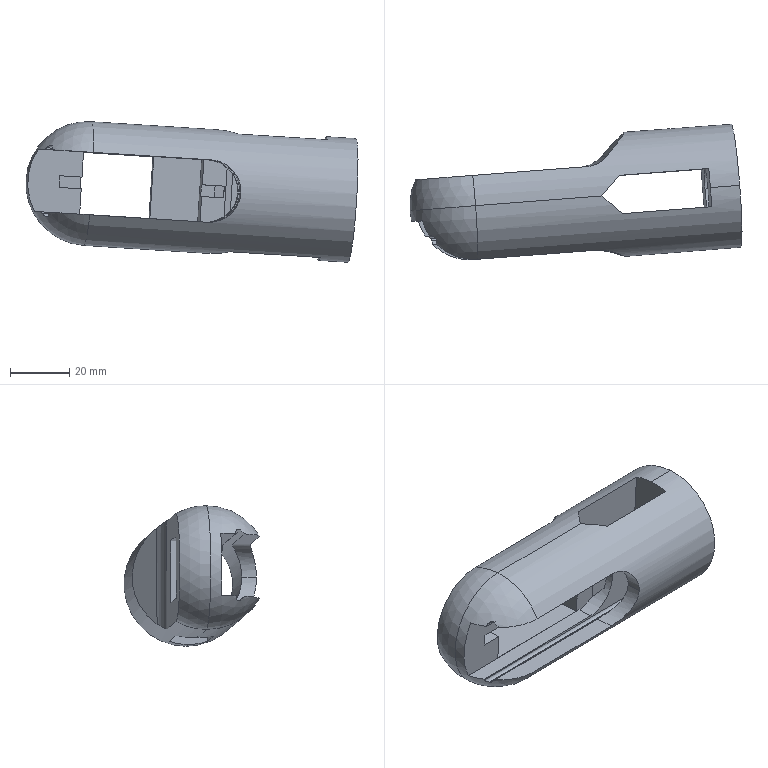Component | SolidWorks | Brazo-06-SW-1 | 1 solid | 46 faces | box 112.64 x 46.02 x 47.67 mm | volume 69156 mm3 | plane 31 | cylinder 13 | sphere 2 | commonest cylinder face diameters 21.2 x4 2 x3 16 x2 42 x2 32 x1 20 x1
build123d program:
from build123d import *

# Parameters (mm, degrees)
SKETCH1_R           = 21
BOSS_EXTRUDE1_DEPTH = 111
FILLET1_R           = 21
SKETCH2_W           = 21
SKETCH2_H           = 24.7
CUT_EXTRUDE1_DEPTH  = 55.5
CUT_EXTRUDE2_DEPTH  = 55.5
CUT_EXTRUDE3_DEPTH  = 115.904
FILLET2_R           = 10
SKETCH5_R           = 8
CUT_EXTRUDE4_DEPTH  = 10
CUT_EXTRUDE7_DEPTH  = 26
SKETCH7_W           = 21.1
SKETCH7_H           = 41
CUT_EXTRUDE8_DEPTH  = 10
SKETCH9_W           = 4
SKETCH9_H           = 56
CUT_EXTRUDE9_DEPTH  = 4


with BuildPart() as part:
    # Sketch1 → Boss-Extrude1 (new body)
    with BuildSketch(Plane.XY):
        Circle(SKETCH1_R)
    extrude(amount=BOSS_EXTRUDE1_DEPTH)

    # Fillet1
    fillet1_edges = [part.edges().sort_by_distance(p)[0] for p in [
        (-21, 0, 111),
    ]]
    fillet(fillet1_edges, radius=FILLET1_R)

    # Sketch2 → Cut-Extrude1 (cut, symmetric)
    with BuildSketch(Plane(origin=(0, 0, 0), x_dir=(1, 0, 0), z_dir=(0, 1, 0))):
        with Locations((0, -80)):
            Rectangle(SKETCH2_W, SKETCH2_H)
    extrude(amount=CUT_EXTRUDE1_DEPTH, both=True, mode=Mode.SUBTRACT)

    # Sketch3 → Cut-Extrude2 (cut, symmetric)
    with BuildSketch(Plane(origin=(0, 0, 0), x_dir=(0, 0, -1), z_dir=(1, 0, 0))):
        Polygon((-36.3, 21), (-47, 10.3), (-116.459, 10.3), (-116.459, 21), align=None)
        Polygon((-10, 6.5), (-10, -6.5), (-40.5, -6.5), (-47, 0), (-40.5, 6.5), align=None)
    extrude(amount=CUT_EXTRUDE2_DEPTH, both=True, mode=Mode.SUBTRACT)

    # Sketch4 → Cut-Extrude3 (cut, through all)
    with BuildSketch(Plane(origin=(0, 0, 0), x_dir=(-1, 0, 0), z_dir=(0, 0, -1))):
        with BuildLine():
            Line((-11.18, -9), (11.18, -9))
            ThreePointArc((11.18, -9), (12.093, -9.592), (11.926, -10.667))
            ThreePointArc((11.926, -10.667), (0, -16), (-11.926, -10.667))
            ThreePointArc((-11.926, -10.667), (-12.093, -9.592), (-11.18, -9))
        make_face()
    extrude(amount=-CUT_EXTRUDE3_DEPTH, mode=Mode.SUBTRACT)

    # Fillet2
    fillet2_edges = [part.edges().sort_by_distance(p)[0] for p in [
        (0, 10.3, 47),
    ]]
    fillet(fillet2_edges, radius=FILLET2_R)

    # Sketch5 → Cut-Extrude4 (cut)
    with BuildSketch(Plane(origin=(0, 0, 0), x_dir=(-1, 0, 0), z_dir=(0, 0, -1))):
        Circle(SKETCH5_R)
    extrude(amount=-CUT_EXTRUDE4_DEPTH, mode=Mode.SUBTRACT)

    # Sketch6 → Cut-Extrude7 (cut)
    with BuildSketch(Plane(origin=(0, -29.7, 0), x_dir=(1, 0, 0), z_dir=(0, 1, 0))):
        with BuildLine():
            Line((10.6, -50), (10.6, -123.464))
            ThreePointArc((10.6, -123.464), (0, -134.064), (-10.6, -123.464))
            Line((-10.6, -123.464), (-10.6, -50))
            ThreePointArc((-10.6, -50), (0, -39.4), (10.6, -50))
        make_face()
    extrude(amount=CUT_EXTRUDE7_DEPTH, mode=Mode.SUBTRACT)

    # Sketch7 → Cut-Extrude8 (cut)
    with BuildSketch(Plane.XZ.offset(3.7)):
        with Locations((0.05, 71.85)):
            Rectangle(SKETCH7_W, SKETCH7_H)
    extrude(amount=-CUT_EXTRUDE8_DEPTH, mode=Mode.SUBTRACT)

    # Sketch9 → Cut-Extrude9 (cut)
    with BuildSketch(Plane.XZ.offset(3.7)):
        with Locations((0.05, 71.85)):
            Rectangle(SKETCH9_W, SKETCH9_H)
    extrude(amount=-CUT_EXTRUDE9_DEPTH, mode=Mode.SUBTRACT)


solid = part.part

# Placed as in the assembly
solid = solid.moved(Location((37.37, -46.285, 824.227), (50.389, -84.291, 50.529)))